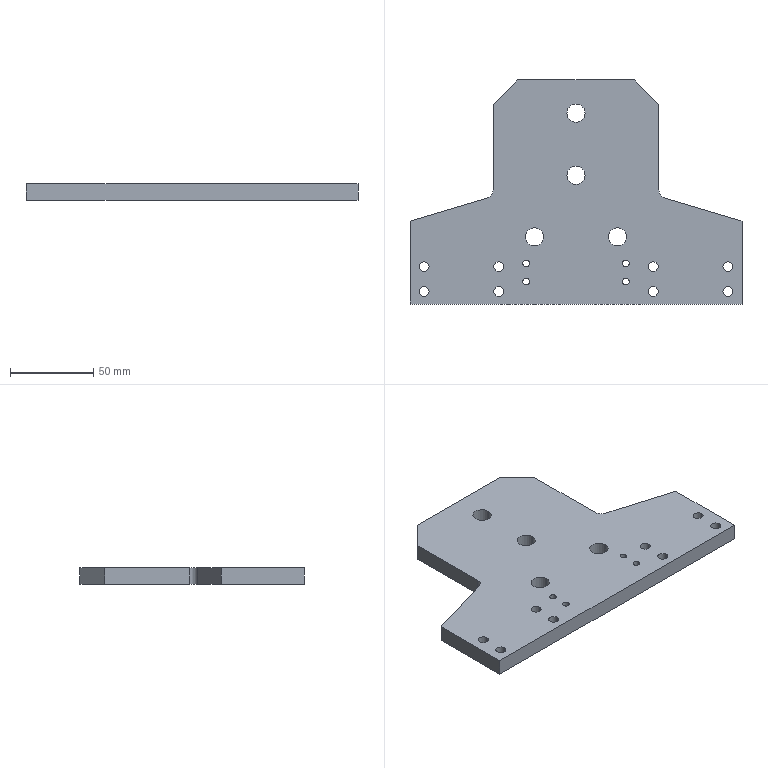Component | SolidWorks | Yk1.5.1AttachmentPlate-1 | 1 solid | 46 faces | volume 183736 mm3 | cylinder 34 | plane 12 | commonest cylinder face diameters 6 x16 4 x8 11 x8 10 x2 | material Q235B